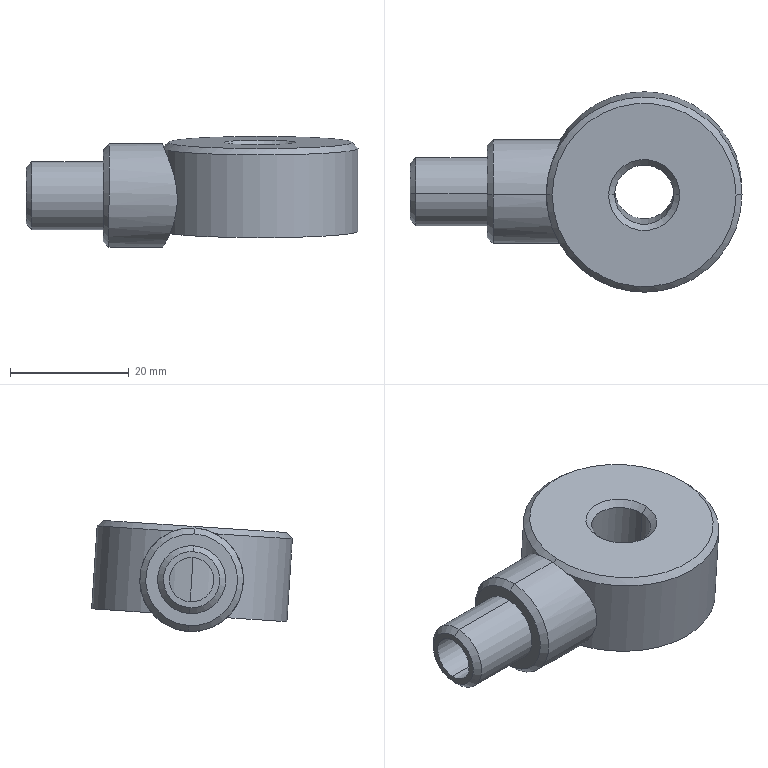Component | SolidWorks | LEDAlarm-1_UpperRotatingHead-1 | 3 solids | 27 faces | box 56 x 33.85 x 18.75 mm | volume 13801 mm3 | cylinder 14 | cone 8 | plane 5 | commonest cylinder face diameters 11.5 x4 33 x4 7.5 x2 17.5 x2 10 x2
build123d program:
from build123d import *

# Parameters (mm, degrees)
SKETCH1_R                = 16.5
SKETCH1_R_2              = 5
BOSS_EXTRUDE1_DEPTH      = 15
CHAMFER1_SIZE            = 1
EXTRUDE_THIN1_REACH      = 50.438
EXTRUDE_THIN1_END_RADIUS = 16.5
SKETCH3_R                = 8.75
SKETCH3_R_2              = 5.75
SKETCH4_R                = 5.75
SKETCH4_R_2              = 3.75
EXTRUDE_THIN2_DEPTH      = 13
CHAMFER2_SIZE            = 1
CHAMFER3_SIZE            = 1


with BuildPart() as part:
    # Sketch1 → Boss-Extrude1 (new body)
    with BuildSketch(Plane.XY):
        Circle(SKETCH1_R)
        Circle(SKETCH1_R_2, mode=Mode.SUBTRACT)
    extrude(amount=BOSS_EXTRUDE1_DEPTH)

    # Chamfer1
    chamfer1_edges = [part.edges().sort_by_distance(p)[0] for p in [
        (-16.5, 0, 15),
        (-5, 0, 15),
    ]]
    chamfer(chamfer1_edges, length=CHAMFER1_SIZE)


with BuildPart() as body_2:
    # Extrude-Thin1: up to this cylinder (the profile starts outside it)
    extrude_thin1_end = Plane(origin=(0, 0, -2.503), z_dir=(0, 0, -1)) * Cylinder(EXTRUDE_THIN1_END_RADIUS, 134.876, mode=Mode.PRIVATE)
    # Sketch3 → Extrude-Thin1 (new, up to the surface)
    with BuildSketch(Plane.ZY.offset(26.5), mode=Mode.PRIVATE) as extrude_thin1_sk1:
        with Locations((6, 0)):
            Circle(SKETCH3_R)
        with Locations((6, 0)):
            Circle(SKETCH3_R_2, mode=Mode.SUBTRACT)
    extrude_thin1_tool1 = extrude(extrude_thin1_sk1.sketch, amount=-EXTRUDE_THIN1_REACH, mode=Mode.PRIVATE) - extrude_thin1_end
    add(extrude_thin1_tool1.solids().sort_by_distance((-26.5, 0, -2.503))[0])

    # Chamfer2
    chamfer2_edges = [body_2.edges().sort_by_distance(p)[0] for p in [
        (-26.5, 0, -2.75),
    ]]
    chamfer(chamfer2_edges, length=CHAMFER2_SIZE)


with BuildPart() as body_3:
    # Sketch4 → Extrude-Thin2 (new body)
    with BuildSketch(Plane.ZY.offset(26.5)):
        with Locations((6, 0)):
            Circle(SKETCH4_R)
        with Locations((6, 0)):
            Circle(SKETCH4_R_2, mode=Mode.SUBTRACT)
    extrude(amount=EXTRUDE_THIN2_DEPTH)

    # Chamfer3
    chamfer3_edges = [body_3.edges().sort_by_distance(p)[0] for p in [
        (-39.5, 0, 0.25),
    ]]
    chamfer(chamfer3_edges, length=CHAMFER3_SIZE)


solid = Compound([part.part, body_2.part, body_3.part])

# Placed as in the assembly
solid = solid.moved(Location((826.947, 455.702, 430.35), (3.768, 0.005615, -0.0003082)))
STEP:
#1=CARTESIAN_POINT('',(31.002,17.913,17.365));
#2=VERTEX_POINT('',#1);
#3=CARTESIAN_POINT('',(31.002,17.938,16.992));
#4=VERTEX_POINT('',#3);
#5=CARTESIAN_POINT('',(31.002,17.925,17.179));
#6=DIRECTION('',(-1.,0.,0.00009864));
#7=DIRECTION('',(0.00009843,-0.06571,0.9978));
#8=AXIS2_PLACEMENT_3D('',#5,#6,#7);
#9=CIRCLE('',#8,0.187);
#10=EDGE_CURVE('',#2,#4,#9,.T.);
#11=ORIENTED_EDGE('',*,*,#10,.F.);
#12=CARTESIAN_POINT('',(31.041,17.911,17.405));
#13=VERTEX_POINT('',#12);
#14=CARTESIAN_POINT('',(31.002,17.913,17.365));
#15=DIRECTION('',(0.7072,-0.04647,0.7055));
#16=VECTOR('',#15,39.37);
#17=LINE('',#14,#16);
#18=EDGE_CURVE('',#2,#13,#17,.T.);
#19=ORIENTED_EDGE('',*,*,#18,.T.);
#20=CARTESIAN_POINT('',(31.041,17.94,16.953));
#21=VERTEX_POINT('',#20);
#22=CARTESIAN_POINT('',(31.041,17.925,17.179));
#23=DIRECTION('',(1.,-0.,-0.00009864));
#24=DIRECTION('',(0.00009843,-0.06571,0.9978));
#25=AXIS2_PLACEMENT_3D('',#22,#23,#24);
#26=CIRCLE('',#25,0.2264);
#27=EDGE_CURVE('',#21,#13,#26,.T.);
#28=ORIENTED_EDGE('',*,*,#27,.F.);
#29=CARTESIAN_POINT('',(31.002,17.938,16.992));
#30=DIRECTION('',(0.707,0.04647,-0.7056));
#31=VECTOR('',#30,39.37);
#32=LINE('',#29,#31);
#33=EDGE_CURVE('',#4,#21,#32,.T.);
#34=ORIENTED_EDGE('',*,*,#33,.F.);
#35=EDGE_LOOP('',(#11,#19,#28,#34));
#36=FACE_OUTER_BOUND('',#35,.T.);
#37=CARTESIAN_POINT('',(31.002,17.925,17.179));
#38=DIRECTION('',(1.,-0.,-0.00009864));
#39=DIRECTION('',(-0.00009843,0.06571,-0.9978));
#40=AXIS2_PLACEMENT_3D('',#37,#38,#39);
#41=CONICAL_SURFACE('',#40,0.187,0.7854);
#42=ADVANCED_FACE('',(#36),#41,.T.);
#43=CARTESIAN_POINT('',(31.002,17.935,17.031));
#44=VERTEX_POINT('',#43);
#45=CARTESIAN_POINT('',(31.002,17.916,17.326));
#46=VERTEX_POINT('',#45);
#47=CARTESIAN_POINT('',(31.002,17.925,17.179));
#48=DIRECTION('',(-1.,0.,0.00009864));
#49=DIRECTION('',(0.00009843,-0.06571,0.9978));
#50=AXIS2_PLACEMENT_3D('',#47,#48,#49);
#51=CIRCLE('',#50,0.1476);
#52=EDGE_CURVE('',#44,#46,#51,.T.);
#53=ORIENTED_EDGE('',*,*,#52,.T.);
#54=CARTESIAN_POINT('',(31.514,17.916,17.326));
#55=VERTEX_POINT('',#54);
#56=CARTESIAN_POINT('',(31.002,17.916,17.326));
#57=DIRECTION('',(1.,-0.,-0.00009864));
#58=VECTOR('',#57,39.37);
#59=LINE('',#56,#58);
#60=EDGE_CURVE('',#46,#55,#59,.T.);
#61=ORIENTED_EDGE('',*,*,#60,.T.);
#62=CARTESIAN_POINT('',(31.514,17.935,17.031));
#63=VERTEX_POINT('',#62);
#64=CARTESIAN_POINT('',(31.514,17.925,17.179));
#65=DIRECTION('',(-1.,0.,0.00009864));
#66=DIRECTION('',(0.00009843,-0.06571,0.9978));
#67=AXIS2_PLACEMENT_3D('',#64,#65,#66);
#68=CIRCLE('',#67,0.1476);
#69=EDGE_CURVE('',#63,#55,#68,.T.);
#70=ORIENTED_EDGE('',*,*,#69,.F.);
#71=CARTESIAN_POINT('',(31.002,17.935,17.031));
#72=DIRECTION('',(1.,-0.,-0.00009864));
#73=VECTOR('',#72,39.37);
#74=LINE('',#71,#73);
#75=EDGE_CURVE('',#44,#63,#74,.T.);
#76=ORIENTED_EDGE('',*,*,#75,.F.);
#77=EDGE_LOOP('',(#53,#61,#70,#76));
#78=FACE_OUTER_BOUND('',#77,.T.);
#79=CARTESIAN_POINT('',(31.002,17.925,17.179));
#80=DIRECTION('',(1.,-0.,-0.00009864));
#81=DIRECTION('',(-0.00009843,0.06571,-0.9978));
#82=AXIS2_PLACEMENT_3D('',#79,#80,#81);
#83=CYLINDRICAL_SURFACE('',#82,0.1476);
#84=ADVANCED_FACE('',(#78),#83,.F.);
#85=ORIENTED_EDGE('',*,*,#27,.T.);
#86=CARTESIAN_POINT('',(31.514,17.911,17.405));
#87=VERTEX_POINT('',#86);
#88=CARTESIAN_POINT('',(31.002,17.911,17.405));
#89=DIRECTION('',(1.,-0.,-0.00009864));
#90=VECTOR('',#89,39.37);
#91=LINE('',#88,#90);
#92=EDGE_CURVE('',#13,#87,#91,.T.);
#93=ORIENTED_EDGE('',*,*,#92,.T.);
#94=CARTESIAN_POINT('',(31.514,17.94,16.953));
#95=VERTEX_POINT('',#94);
#96=CARTESIAN_POINT('',(31.514,17.925,17.179));
#97=DIRECTION('',(-1.,0.,0.00009864));
#98=DIRECTION('',(0.00009843,-0.06571,0.9978));
#99=AXIS2_PLACEMENT_3D('',#96,#97,#98);
#100=CIRCLE('',#99,0.2264);
#101=EDGE_CURVE('',#87,#95,#100,.T.);
#102=ORIENTED_EDGE('',*,*,#101,.T.);
#103=CARTESIAN_POINT('',(31.002,17.94,16.953));
#104=DIRECTION('',(1.,-0.,-0.00009864));
#105=VECTOR('',#104,39.37);
#106=LINE('',#103,#105);
#107=EDGE_CURVE('',#21,#95,#106,.T.);
#108=ORIENTED_EDGE('',*,*,#107,.F.);
#109=EDGE_LOOP('',(#85,#93,#102,#108));
#110=FACE_OUTER_BOUND('',#109,.T.);
#111=CARTESIAN_POINT('',(31.002,17.925,17.179));
#112=DIRECTION('',(1.,-0.,-0.00009864));
#113=DIRECTION('',(-0.00009843,0.06571,-0.9978));
#114=AXIS2_PLACEMENT_3D('',#111,#112,#113);
#115=CYLINDRICAL_SURFACE('',#114,0.2264);
#116=ADVANCED_FACE('',(#110),#115,.T.);
#117=CARTESIAN_POINT('',(31.002,17.925,17.179));
#118=DIRECTION('',(-1.,0.,0.00009864));
#119=DIRECTION('',(0.00009843,-0.06571,0.9978));
#120=AXIS2_PLACEMENT_3D('',#117,#118,#119);
#121=CIRCLE('',#120,0.187);
#122=EDGE_CURVE('',#4,#2,#121,.T.);
#123=ORIENTED_EDGE('',*,*,#122,.T.);
#124=ORIENTED_EDGE('',*,*,#10,.T.);
#125=EDGE_LOOP('',(#123,#124));
#126=FACE_OUTER_BOUND('',#125,.T.);
#127=ORIENTED_EDGE('',*,*,#52,.F.);
#128=CARTESIAN_POINT('',(31.002,17.925,17.179));
#129=DIRECTION('',(-1.,0.,0.00009864));
#130=DIRECTION('',(0.00009843,-0.06571,0.9978));
#131=AXIS2_PLACEMENT_3D('',#128,#129,#130);
#132=CIRCLE('',#131,0.1476);
#133=EDGE_CURVE('',#46,#44,#132,.T.);
#134=ORIENTED_EDGE('',*,*,#133,.F.);
#135=EDGE_LOOP('',(#127,#134));
#136=FACE_BOUND('',#135,.T.);
#137=CARTESIAN_POINT('',(31.002,17.925,17.179));
#138=DIRECTION('',(-1.,0.,0.00009864));
#139=DIRECTION('',(0.00009843,-0.06571,0.9978));
#140=AXIS2_PLACEMENT_3D('',#137,#138,#139);
#141=PLANE('',#140);
#142=ADVANCED_FACE('',(#126,#136),#141,.T.);
#143=CARTESIAN_POINT('',(31.514,17.925,17.179));
#144=DIRECTION('',(-1.,0.,0.00009864));
#145=DIRECTION('',(0.00009843,-0.06571,0.9978));
#146=AXIS2_PLACEMENT_3D('',#143,#144,#145);
#147=CIRCLE('',#146,0.2264);
#148=EDGE_CURVE('',#95,#87,#147,.T.);
#149=ORIENTED_EDGE('',*,*,#148,.F.);
#150=ORIENTED_EDGE('',*,*,#101,.F.);
#151=EDGE_LOOP('',(#149,#150));
#152=FACE_OUTER_BOUND('',#151,.T.);
#153=ORIENTED_EDGE('',*,*,#69,.T.);
#154=CARTESIAN_POINT('',(31.514,17.925,17.179));
#155=DIRECTION('',(-1.,0.,0.00009864));
#156=DIRECTION('',(0.00009843,-0.06571,0.9978));
#157=AXIS2_PLACEMENT_3D('',#154,#155,#156);
#158=CIRCLE('',#157,0.1476);
#159=EDGE_CURVE('',#55,#63,#158,.T.);
#160=ORIENTED_EDGE('',*,*,#159,.T.);
#161=EDGE_LOOP('',(#153,#160));
#162=FACE_BOUND('',#161,.T.);
#163=CARTESIAN_POINT('',(31.514,17.925,17.179));
#164=DIRECTION('',(-1.,0.,0.00009864));
#165=DIRECTION('',(0.00009843,-0.06571,0.9978));
#166=AXIS2_PLACEMENT_3D('',#163,#164,#165);
#167=PLANE('',#166);
#168=ADVANCED_FACE('',(#152,#162),#167,.F.);
#169=ORIENTED_EDGE('',*,*,#92,.F.);
#170=CARTESIAN_POINT('',(31.041,17.925,17.179));
#171=DIRECTION('',(1.,-0.,-0.00009864));
#172=DIRECTION('',(0.00009843,-0.06571,0.9978));
#173=AXIS2_PLACEMENT_3D('',#170,#171,#172);
#174=CIRCLE('',#173,0.2264);
#175=EDGE_CURVE('',#13,#21,#174,.T.);
#176=ORIENTED_EDGE('',*,*,#175,.T.);
#177=ORIENTED_EDGE('',*,*,#107,.T.);
#178=ORIENTED_EDGE('',*,*,#148,.T.);
#179=EDGE_LOOP('',(#169,#176,#177,#178));
#180=FACE_OUTER_BOUND('',#179,.T.);
#181=CARTESIAN_POINT('',(31.002,17.925,17.179));
#182=DIRECTION('',(1.,-0.,-0.00009864));
#183=DIRECTION('',(-0.00009843,0.06571,-0.9978));
#184=AXIS2_PLACEMENT_3D('',#181,#182,#183);
#185=CYLINDRICAL_SURFACE('',#184,0.2264);
#186=ADVANCED_FACE('',(#180),#185,.T.);
#187=ORIENTED_EDGE('',*,*,#60,.F.);
#188=ORIENTED_EDGE('',*,*,#133,.T.);
#189=ORIENTED_EDGE('',*,*,#75,.T.);
#190=ORIENTED_EDGE('',*,*,#159,.F.);
#191=EDGE_LOOP('',(#187,#188,#189,#190));
#192=FACE_OUTER_BOUND('',#191,.T.);
#193=CARTESIAN_POINT('',(31.002,17.925,17.179));
#194=DIRECTION('',(1.,-0.,-0.00009864));
#195=DIRECTION('',(-0.00009843,0.06571,-0.9978));
#196=AXIS2_PLACEMENT_3D('',#193,#194,#195);
#197=CYLINDRICAL_SURFACE('',#196,0.1476);
#198=ADVANCED_FACE('',(#192),#197,.F.);
#199=ORIENTED_EDGE('',*,*,#18,.F.);
#200=ORIENTED_EDGE('',*,*,#122,.F.);
#201=ORIENTED_EDGE('',*,*,#33,.T.);
#202=ORIENTED_EDGE('',*,*,#175,.F.);
#203=EDGE_LOOP('',(#199,#200,#201,#202));
#204=FACE_OUTER_BOUND('',#203,.T.);
#205=CARTESIAN_POINT('',(31.002,17.925,17.179));
#206=DIRECTION('',(1.,-0.,-0.00009864));
#207=DIRECTION('',(-0.00009843,0.06571,-0.9978));
#208=AXIS2_PLACEMENT_3D('',#205,#206,#207);
#209=CONICAL_SURFACE('',#208,0.187,0.7854);
#210=ADVANCED_FACE('',(#204),#209,.T.);
#211=CLOSED_SHELL('',(#42,#84,#116,#142,#168,#186,#198,#210));
#212=MANIFOLD_SOLID_BREP('',#211);
#213=CARTESIAN_POINT('',(31.514,17.905,17.483));
#214=VERTEX_POINT('',#213);
#215=CARTESIAN_POINT('',(31.514,17.946,16.874));
#216=VERTEX_POINT('',#215);
#217=CARTESIAN_POINT('',(31.514,17.925,17.179));
#218=DIRECTION('',(-1.,0.,0.00009864));
#219=DIRECTION('',(0.00009843,-0.06571,0.9978));
#220=AXIS2_PLACEMENT_3D('',#217,#218,#219);
#221=CIRCLE('',#220,0.3051);
#222=EDGE_CURVE('',#214,#216,#221,.T.);
#223=ORIENTED_EDGE('',*,*,#222,.F.);
#224=CARTESIAN_POINT('',(31.553,17.903,17.522));
#225=VERTEX_POINT('',#224);
#226=CARTESIAN_POINT('',(31.514,17.905,17.483));
#227=DIRECTION('',(0.7072,-0.04647,0.7055));
#228=VECTOR('',#227,39.37);
#229=LINE('',#226,#228);
#230=EDGE_CURVE('',#214,#225,#229,.T.);
#231=ORIENTED_EDGE('',*,*,#230,.T.);
#232=CARTESIAN_POINT('',(31.553,17.948,16.835));
#233=VERTEX_POINT('',#232);
#234=CARTESIAN_POINT('',(31.553,17.925,17.179));
#235=DIRECTION('',(1.,-0.,-0.00009864));
#236=DIRECTION('',(0.00009843,-0.06571,0.9978));
#237=AXIS2_PLACEMENT_3D('',#234,#235,#236);
#238=CIRCLE('',#237,0.3445);
#239=EDGE_CURVE('',#233,#225,#238,.T.);
#240=ORIENTED_EDGE('',*,*,#239,.F.);
#241=CARTESIAN_POINT('',(31.514,17.946,16.874));
#242=DIRECTION('',(0.707,0.04647,-0.7056));
#243=VECTOR('',#242,39.37);
#244=LINE('',#241,#243);
#245=EDGE_CURVE('',#216,#233,#244,.T.);
#246=ORIENTED_EDGE('',*,*,#245,.F.);
#247=EDGE_LOOP('',(#223,#231,#240,#246));
#248=FACE_OUTER_BOUND('',#247,.T.);
#249=CARTESIAN_POINT('',(31.514,17.925,17.179));
#250=DIRECTION('',(1.,-0.,-0.00009864));
#251=DIRECTION('',(-0.00009843,0.06571,-0.9978));
#252=AXIS2_PLACEMENT_3D('',#249,#250,#251);
#253=CONICAL_SURFACE('',#252,0.3051,0.7854);
#254=ADVANCED_FACE('',(#248),#253,.T.);
#255=CARTESIAN_POINT('',(31.907,17.94,16.953));
#256=VERTEX_POINT('',#255);
#257=CARTESIAN_POINT('',(31.907,17.911,17.405));
#258=VERTEX_POINT('',#257);
#259=CARTESIAN_POINT('',(31.907,17.94,16.953));
#260=CARTESIAN_POINT('',(31.907,17.933,16.952));
#261=CARTESIAN_POINT('',(31.908,17.926,16.952));
#262=CARTESIAN_POINT('',(31.908,17.911,16.953));
#263=CARTESIAN_POINT('',(31.908,17.903,16.953));
#264=CARTESIAN_POINT('',(31.91,17.881,16.956));
#265=CARTESIAN_POINT('',(31.911,17.866,16.96));
#266=CARTESIAN_POINT('',(31.915,17.838,16.969));
#267=CARTESIAN_POINT('',(31.917,17.825,16.975));
#268=CARTESIAN_POINT('',(31.922,17.799,16.99));
#269=CARTESIAN_POINT('',(31.925,17.787,16.999));
#270=CARTESIAN_POINT('',(31.93,17.765,17.018));
#271=CARTESIAN_POINT('',(31.933,17.755,17.029));
#272=CARTESIAN_POINT('',(31.936,17.742,17.046));
#273=CARTESIAN_POINT('',(31.938,17.737,17.052));
#274=CARTESIAN_POINT('',(31.94,17.73,17.065));
#275=CARTESIAN_POINT('',(31.941,17.726,17.072));
#276=CARTESIAN_POINT('',(31.944,17.716,17.092));
#277=CARTESIAN_POINT('',(31.945,17.711,17.105));
#278=CARTESIAN_POINT('',(31.948,17.703,17.134));
#279=CARTESIAN_POINT('',(31.948,17.701,17.149));
#280=CARTESIAN_POINT('',(31.948,17.699,17.179));
#281=CARTESIAN_POINT('',(31.948,17.699,17.194));
#282=CARTESIAN_POINT('',(31.946,17.702,17.216));
#283=CARTESIAN_POINT('',(31.945,17.703,17.223));
#284=CARTESIAN_POINT('',(31.944,17.707,17.238));
#285=CARTESIAN_POINT('',(31.943,17.709,17.245));
#286=CARTESIAN_POINT('',(31.941,17.714,17.259));
#287=CARTESIAN_POINT('',(31.94,17.716,17.266));
#288=CARTESIAN_POINT('',(31.938,17.722,17.279));
#289=CARTESIAN_POINT('',(31.936,17.726,17.286));
#290=CARTESIAN_POINT('',(31.933,17.737,17.305));
#291=CARTESIAN_POINT('',(31.93,17.746,17.317));
#292=CARTESIAN_POINT('',(31.925,17.765,17.339));
#293=CARTESIAN_POINT('',(31.922,17.776,17.349));
#294=CARTESIAN_POINT('',(31.917,17.799,17.367));
#295=CARTESIAN_POINT('',(31.915,17.812,17.375));
#296=CARTESIAN_POINT('',(31.912,17.832,17.385));
#297=CARTESIAN_POINT('',(31.912,17.838,17.388));
#298=CARTESIAN_POINT('',(31.91,17.852,17.393));
#299=CARTESIAN_POINT('',(31.909,17.859,17.395));
#300=CARTESIAN_POINT('',(31.908,17.881,17.401));
#301=CARTESIAN_POINT('',(31.907,17.896,17.404));
#302=CARTESIAN_POINT('',(31.907,17.911,17.405));
#303=B_SPLINE_CURVE_WITH_KNOTS('',3,(#259,#260,#261,#262,#263,#264,#265,#266,#267,#268,#269,#270,#271,#272,#273,#274,#275,#276,#277,#278,#279,#280,#281,#282,#283,#284,#285,#286,#287,#288,#289,#290,#291,#292,#293,#294,#295,#296,#297,#298,#299,#300,#301,#302),.UNSPECIFIED.,.F.,.F.,(4,2,2,2,2,2,2,2,2,2,2,2,2,2,2,2,2,2,2,2,2,4),(0.01812,0.01869,0.01925,0.02038,0.02152,0.02265,0.02378,0.02435,0.02491,0.02605,0.02718,0.02831,0.02888,0.02944,0.03001,0.03058,0.03171,0.03284,0.03397,0.03454,0.0351,0.03624),.UNSPECIFIED.);
#304=EDGE_CURVE('',#256,#258,#303,.T.);
#305=ORIENTED_EDGE('',*,*,#304,.F.);
#306=CARTESIAN_POINT('',(31.514,17.94,16.953));
#307=VERTEX_POINT('',#306);
#308=CARTESIAN_POINT('',(33.207,17.94,16.953));
#309=DIRECTION('',(-1.,0.,0.00009864));
#310=VECTOR('',#309,39.37);
#311=LINE('',#308,#310);
#312=EDGE_CURVE('',#256,#307,#311,.T.);
#313=ORIENTED_EDGE('',*,*,#312,.T.);
#314=CARTESIAN_POINT('',(31.514,17.911,17.405));
#315=VERTEX_POINT('',#314);
#316=CARTESIAN_POINT('',(31.514,17.925,17.179));
#317=DIRECTION('',(-1.,0.,0.00009864));
#318=DIRECTION('',(0.00009843,-0.06571,0.9978));
#319=AXIS2_PLACEMENT_3D('',#316,#317,#318);
#320=CIRCLE('',#319,0.2264);
#321=EDGE_CURVE('',#307,#315,#320,.T.);
#322=ORIENTED_EDGE('',*,*,#321,.T.);
#323=CARTESIAN_POINT('',(33.207,17.911,17.404));
#324=DIRECTION('',(-1.,0.,0.00009864));
#325=VECTOR('',#324,39.37);
#326=LINE('',#323,#325);
#327=EDGE_CURVE('',#258,#315,#326,.T.);
#328=ORIENTED_EDGE('',*,*,#327,.F.);
#329=EDGE_LOOP('',(#305,#313,#322,#328));
#330=FACE_OUTER_BOUND('',#329,.T.);
#331=CARTESIAN_POINT('',(33.207,17.925,17.179));
#332=DIRECTION('',(-1.,0.,0.00009864));
#333=DIRECTION('',(0.00009843,-0.06571,0.9978));
#334=AXIS2_PLACEMENT_3D('',#331,#332,#333);
#335=CYLINDRICAL_SURFACE('',#334,0.2264);
#336=ADVANCED_FACE('',(#330),#335,.F.);
#337=CARTESIAN_POINT('',(31.907,17.903,17.522));
#338=VERTEX_POINT('',#337);
#339=CARTESIAN_POINT('',(31.907,17.948,16.835));
#340=VERTEX_POINT('',#339);
#341=CARTESIAN_POINT('',(31.907,17.903,17.522));
#342=CARTESIAN_POINT('',(31.907,17.926,17.524));
#343=CARTESIAN_POINT('',(31.909,17.949,17.523));
#344=CARTESIAN_POINT('',(31.913,17.994,17.517));
#345=CARTESIAN_POINT('',(31.917,18.017,17.512));
#346=CARTESIAN_POINT('',(31.926,18.059,17.497));
#347=CARTESIAN_POINT('',(31.931,18.08,17.488));
#348=CARTESIAN_POINT('',(31.94,18.109,17.471));
#349=CARTESIAN_POINT('',(31.943,18.118,17.465));
#350=CARTESIAN_POINT('',(31.949,18.136,17.452));
#351=CARTESIAN_POINT('',(31.952,18.145,17.445));
#352=CARTESIAN_POINT('',(31.958,18.161,17.43));
#353=CARTESIAN_POINT('',(31.961,18.169,17.423));
#354=CARTESIAN_POINT('',(31.968,18.184,17.406));
#355=CARTESIAN_POINT('',(31.971,18.192,17.398));
#356=CARTESIAN_POINT('',(31.98,18.212,17.371));
#357=CARTESIAN_POINT('',(31.986,18.224,17.353));
#358=CARTESIAN_POINT('',(31.993,18.239,17.323));
#359=CARTESIAN_POINT('',(31.995,18.243,17.312));
#360=CARTESIAN_POINT('',(31.999,18.251,17.291));
#361=CARTESIAN_POINT('',(32.001,18.255,17.28));
#362=CARTESIAN_POINT('',(32.005,18.264,17.247));
#363=CARTESIAN_POINT('',(32.006,18.268,17.225));
#364=CARTESIAN_POINT('',(32.006,18.27,17.19));
#365=CARTESIAN_POINT('',(32.006,18.27,17.179));
#366=CARTESIAN_POINT('',(32.004,18.269,17.156));
#367=CARTESIAN_POINT('',(32.003,18.268,17.144));
#368=CARTESIAN_POINT('',(32.001,18.265,17.122));
#369=CARTESIAN_POINT('',(31.999,18.263,17.11));
#370=CARTESIAN_POINT('',(31.995,18.258,17.088));
#371=CARTESIAN_POINT('',(31.993,18.255,17.077));
#372=CARTESIAN_POINT('',(31.985,18.244,17.045));
#373=CARTESIAN_POINT('',(31.98,18.235,17.025));
#374=CARTESIAN_POINT('',(31.971,18.218,16.996));
#375=CARTESIAN_POINT('',(31.967,18.212,16.987));
#376=CARTESIAN_POINT('',(31.961,18.199,16.969));
#377=CARTESIAN_POINT('',(31.958,18.192,16.96));
#378=CARTESIAN_POINT('',(31.949,18.17,16.935));
#379=CARTESIAN_POINT('',(31.942,18.154,16.92));
#380=CARTESIAN_POINT('',(31.931,18.118,16.892));
#381=CARTESIAN_POINT('',(31.926,18.1,16.881));
#382=CARTESIAN_POINT('',(31.919,18.069,16.866));
#383=CARTESIAN_POINT('',(31.917,18.059,16.861));
#384=CARTESIAN_POINT('',(31.914,18.038,16.853));
#385=CARTESIAN_POINT('',(31.912,18.027,16.849));
#386=CARTESIAN_POINT('',(31.909,17.994,16.84));
#387=CARTESIAN_POINT('',(31.907,17.971,16.836));
#388=CARTESIAN_POINT('',(31.907,17.948,16.835));
#389=B_SPLINE_CURVE_WITH_KNOTS('',3,(#341,#342,#343,#344,#345,#346,#347,#348,#349,#350,#351,#352,#353,#354,#355,#356,#357,#358,#359,#360,#361,#362,#363,#364,#365,#366,#367,#368,#369,#370,#371,#372,#373,#374,#375,#376,#377,#378,#379,#380,#381,#382,#383,#384,#385,#386,#387,#388),.UNSPECIFIED.,.F.,.F.,(4,2,2,2,2,2,2,2,2,2,2,2,2,2,2,2,2,2,2,2,2,2,2,4),(0.,0.001744,0.003488,0.005232,0.006103,0.006975,0.007847,0.008719,0.01046,0.01133,0.01221,0.01395,0.01482,0.01569,0.01657,0.01744,0.01918,0.02005,0.02093,0.02267,0.02441,0.02529,0.02616,0.0279),.UNSPECIFIED.);
#390=EDGE_CURVE('',#338,#340,#389,.T.);
#391=ORIENTED_EDGE('',*,*,#390,.T.);
#392=CARTESIAN_POINT('',(33.207,17.948,16.835));
#393=DIRECTION('',(-1.,0.,0.00009864));
#394=VECTOR('',#393,39.37);
#395=LINE('',#392,#394);
#396=EDGE_CURVE('',#340,#233,#395,.T.);
#397=ORIENTED_EDGE('',*,*,#396,.T.);
#398=ORIENTED_EDGE('',*,*,#239,.T.);
#399=CARTESIAN_POINT('',(33.207,17.903,17.522));
#400=DIRECTION('',(-1.,0.,0.00009864));
#401=VECTOR('',#400,39.37);
#402=LINE('',#399,#401);
#403=EDGE_CURVE('',#338,#225,#402,.T.);
#404=ORIENTED_EDGE('',*,*,#403,.F.);
#405=EDGE_LOOP('',(#391,#397,#398,#404));
#406=FACE_OUTER_BOUND('',#405,.T.);
#407=CARTESIAN_POINT('',(33.207,17.925,17.179));
#408=DIRECTION('',(-1.,0.,0.00009864));
#409=DIRECTION('',(0.00009843,-0.06571,0.9978));
#410=AXIS2_PLACEMENT_3D('',#407,#408,#409);
#411=CYLINDRICAL_SURFACE('',#410,0.3445);
#412=ADVANCED_FACE('',(#406),#411,.T.);
#413=ORIENTED_EDGE('',*,*,#390,.F.);
#414=CARTESIAN_POINT('',(31.907,17.902,17.532));
#415=DIRECTION('',(-0.00009843,0.06571,-0.9978));
#416=VECTOR('',#415,39.37);
#417=LINE('',#414,#416);
#418=EDGE_CURVE('',#338,#258,#417,.T.);
#419=ORIENTED_EDGE('',*,*,#418,.T.);
#420=CARTESIAN_POINT('',(31.907,17.911,17.405));
#421=CARTESIAN_POINT('',(31.907,17.926,17.406));
#422=CARTESIAN_POINT('',(31.908,17.941,17.405));
#423=CARTESIAN_POINT('',(31.909,17.963,17.402));
#424=CARTESIAN_POINT('',(31.91,17.97,17.401));
#425=CARTESIAN_POINT('',(31.912,17.984,17.397));
#426=CARTESIAN_POINT('',(31.912,17.992,17.395));
#427=CARTESIAN_POINT('',(31.915,18.013,17.388));
#428=CARTESIAN_POINT('',(31.917,18.026,17.382));
#429=CARTESIAN_POINT('',(31.921,18.045,17.371));
#430=CARTESIAN_POINT('',(31.922,18.052,17.367));
#431=CARTESIAN_POINT('',(31.925,18.064,17.358));
#432=CARTESIAN_POINT('',(31.926,18.069,17.354));
#433=CARTESIAN_POINT('',(31.93,18.086,17.339));
#434=CARTESIAN_POINT('',(31.933,18.096,17.329));
#435=CARTESIAN_POINT('',(31.938,18.114,17.305));
#436=CARTESIAN_POINT('',(31.94,18.122,17.292));
#437=CARTESIAN_POINT('',(31.943,18.132,17.273));
#438=CARTESIAN_POINT('',(31.944,18.135,17.266));
#439=CARTESIAN_POINT('',(31.945,18.14,17.252));
#440=CARTESIAN_POINT('',(31.946,18.142,17.245));
#441=CARTESIAN_POINT('',(31.948,18.148,17.223));
#442=CARTESIAN_POINT('',(31.948,18.15,17.209));
#443=CARTESIAN_POINT('',(31.948,18.152,17.179));
#444=CARTESIAN_POINT('',(31.948,18.152,17.164));
#445=CARTESIAN_POINT('',(31.945,18.148,17.134));
#446=CARTESIAN_POINT('',(31.944,18.145,17.12));
#447=CARTESIAN_POINT('',(31.94,18.135,17.091));
#448=CARTESIAN_POINT('',(31.938,18.129,17.078));
#449=CARTESIAN_POINT('',(31.934,18.118,17.059));
#450=CARTESIAN_POINT('',(31.933,18.114,17.053));
#451=CARTESIAN_POINT('',(31.93,18.105,17.041));
#452=CARTESIAN_POINT('',(31.929,18.101,17.035));
#453=CARTESIAN_POINT('',(31.925,18.086,17.018));
#454=CARTESIAN_POINT('',(31.922,18.075,17.008));
#455=CARTESIAN_POINT('',(31.917,18.052,16.99));
#456=CARTESIAN_POINT('',(31.915,18.039,16.982));
#457=CARTESIAN_POINT('',(31.911,18.013,16.969));
#458=CARTESIAN_POINT('',(31.91,17.999,16.964));
#459=CARTESIAN_POINT('',(31.908,17.977,16.958));
#460=CARTESIAN_POINT('',(31.908,17.97,16.957));
#461=CARTESIAN_POINT('',(31.908,17.955,16.954));
#462=CARTESIAN_POINT('',(31.907,17.948,16.953));
#463=CARTESIAN_POINT('',(31.907,17.94,16.953));
#464=B_SPLINE_CURVE_WITH_KNOTS('',3,(#420,#421,#422,#423,#424,#425,#426,#427,#428,#429,#430,#431,#432,#433,#434,#435,#436,#437,#438,#439,#440,#441,#442,#443,#444,#445,#446,#447,#448,#449,#450,#451,#452,#453,#454,#455,#456,#457,#458,#459,#460,#461,#462,#463),.UNSPECIFIED.,.F.,.F.,(4,2,2,2,2,2,2,2,2,2,2,2,2,2,2,2,2,2,2,2,2,4),(0.,0.001133,0.001699,0.002265,0.003398,0.003964,0.00453,0.005663,0.006795,0.007361,0.007928,0.00906,0.01019,0.01133,0.01246,0.01302,0.01359,0.01472,0.01586,0.01699,0.01755,0.01812),.UNSPECIFIED.);
#465=EDGE_CURVE('',#258,#256,#464,.T.);
#466=ORIENTED_EDGE('',*,*,#465,.T.);
#467=CARTESIAN_POINT('',(31.907,17.902,17.532));
#468=DIRECTION('',(-0.00009843,0.06571,-0.9978));
#469=VECTOR('',#468,39.37);
#470=LINE('',#467,#469);
#471=EDGE_CURVE('',#256,#340,#470,.T.);
#472=ORIENTED_EDGE('',*,*,#471,.T.);
#473=EDGE_LOOP('',(#413,#419,#466,#472));
#474=FACE_OUTER_BOUND('',#473,.T.);
#475=CARTESIAN_POINT('',(32.557,17.902,17.532));
#476=DIRECTION('',(-0.00009843,0.06571,-0.9978));
#477=DIRECTION('',(-1.,0.,0.00009864));
#478=AXIS2_PLACEMENT_3D('',#475,#476,#477);
#479=CYLINDRICAL_SURFACE('',#478,0.6496);
#480=ADVANCED_FACE('',(#474),#479,.F.);
#481=ORIENTED_EDGE('',*,*,#418,.F.);
#482=CARTESIAN_POINT('',(31.907,17.948,16.835));
#483=CARTESIAN_POINT('',(31.907,17.937,16.834));
#484=CARTESIAN_POINT('',(31.908,17.925,16.834));
#485=CARTESIAN_POINT('',(31.909,17.902,16.835));
#486=CARTESIAN_POINT('',(31.91,17.891,16.836));
#487=CARTESIAN_POINT('',(31.913,17.857,16.84));
#488=CARTESIAN_POINT('',(31.917,17.835,16.846));
#489=CARTESIAN_POINT('',(31.926,17.792,16.86));
#490=CARTESIAN_POINT('',(31.931,17.771,16.87));
#491=CARTESIAN_POINT('',(31.942,17.733,16.892));
#492=CARTESIAN_POINT('',(31.949,17.715,16.905));
#493=CARTESIAN_POINT('',(31.961,17.681,16.935));
#494=CARTESIAN_POINT('',(31.968,17.666,16.951));
#495=CARTESIAN_POINT('',(31.977,17.646,16.977));
#496=CARTESIAN_POINT('',(31.98,17.64,16.986));
#497=CARTESIAN_POINT('',(31.985,17.628,17.005));
#498=CARTESIAN_POINT('',(31.988,17.622,17.015));
#499=CARTESIAN_POINT('',(31.995,17.607,17.045));
#500=CARTESIAN_POINT('',(31.999,17.599,17.066));
#501=CARTESIAN_POINT('',(32.005,17.587,17.11));
#502=CARTESIAN_POINT('',(32.006,17.583,17.133));
#503=CARTESIAN_POINT('',(32.006,17.581,17.167));
#504=CARTESIAN_POINT('',(32.006,17.581,17.178));
#505=CARTESIAN_POINT('',(32.005,17.582,17.201));
#506=CARTESIAN_POINT('',(32.003,17.583,17.213));
#507=CARTESIAN_POINT('',(31.999,17.587,17.247));
#508=CARTESIAN_POINT('',(31.995,17.592,17.269));
#509=CARTESIAN_POINT('',(31.988,17.603,17.301));
#510=CARTESIAN_POINT('',(31.985,17.607,17.312));
#511=CARTESIAN_POINT('',(31.98,17.617,17.332));
#512=CARTESIAN_POINT('',(31.977,17.622,17.342));
#513=CARTESIAN_POINT('',(31.971,17.633,17.361));
#514=CARTESIAN_POINT('',(31.968,17.639,17.37));
#515=CARTESIAN_POINT('',(31.961,17.652,17.388));
#516=CARTESIAN_POINT('',(31.958,17.659,17.397));
#517=CARTESIAN_POINT('',(31.949,17.681,17.422));
#518=CARTESIAN_POINT('',(31.942,17.697,17.437));
#519=CARTESIAN_POINT('',(31.934,17.723,17.458));
#520=CARTESIAN_POINT('',(31.931,17.732,17.464));
#521=CARTESIAN_POINT('',(31.926,17.751,17.476));
#522=CARTESIAN_POINT('',(31.924,17.761,17.482));
#523=CARTESIAN_POINT('',(31.917,17.791,17.497));
#524=CARTESIAN_POINT('',(31.914,17.812,17.505));
#525=CARTESIAN_POINT('',(31.91,17.846,17.514));
#526=CARTESIAN_POINT('',(31.909,17.857,17.516));
#527=CARTESIAN_POINT('',(31.908,17.88,17.52));
#528=CARTESIAN_POINT('',(31.907,17.891,17.522));
#529=CARTESIAN_POINT('',(31.907,17.903,17.522));
#530=B_SPLINE_CURVE_WITH_KNOTS('',3,(#482,#483,#484,#485,#486,#487,#488,#489,#490,#491,#492,#493,#494,#495,#496,#497,#498,#499,#500,#501,#502,#503,#504,#505,#506,#507,#508,#509,#510,#511,#512,#513,#514,#515,#516,#517,#518,#519,#520,#521,#522,#523,#524,#525,#526,#527,#528,#529),.UNSPECIFIED.,.F.,.F.,(4,2,2,2,2,2,2,2,2,2,2,2,2,2,2,2,2,2,2,2,2,2,2,4),(0.0279,0.02877,0.02964,0.03138,0.03312,0.03486,0.0366,0.03747,0.03834,0.04008,0.04182,0.04269,0.04356,0.0453,0.04617,0.04704,0.04791,0.04878,0.05052,0.05139,0.05226,0.054,0.05487,0.05574),.UNSPECIFIED.);
#531=EDGE_CURVE('',#340,#338,#530,.T.);
#532=ORIENTED_EDGE('',*,*,#531,.F.);
#533=ORIENTED_EDGE('',*,*,#471,.F.);
#534=ORIENTED_EDGE('',*,*,#304,.T.);
#535=EDGE_LOOP('',(#481,#532,#533,#534));
#536=FACE_OUTER_BOUND('',#535,.T.);
#537=CARTESIAN_POINT('',(32.557,17.902,17.532));
#538=DIRECTION('',(-0.00009843,0.06571,-0.9978));
#539=DIRECTION('',(-1.,0.,0.00009864));
#540=AXIS2_PLACEMENT_3D('',#537,#538,#539);
#541=CYLINDRICAL_SURFACE('',#540,0.6496);
#542=ADVANCED_FACE('',(#536),#541,.F.);
#543=ORIENTED_EDGE('',*,*,#396,.F.);
#544=ORIENTED_EDGE('',*,*,#531,.T.);
#545=ORIENTED_EDGE('',*,*,#403,.T.);
#546=CARTESIAN_POINT('',(31.553,17.925,17.179));
#547=DIRECTION('',(1.,-0.,-0.00009864));
#548=DIRECTION('',(0.00009843,-0.06571,0.9978));
#549=AXIS2_PLACEMENT_3D('',#546,#547,#548);
#550=CIRCLE('',#549,0.3445);
#551=EDGE_CURVE('',#225,#233,#550,.T.);
#552=ORIENTED_EDGE('',*,*,#551,.T.);
#553=EDGE_LOOP('',(#543,#544,#545,#552));
#554=FACE_OUTER_BOUND('',#553,.T.);
#555=CARTESIAN_POINT('',(33.207,17.925,17.179));
#556=DIRECTION('',(-1.,0.,0.00009864));
#557=DIRECTION('',(0.00009843,-0.06571,0.9978));
#558=AXIS2_PLACEMENT_3D('',#555,#556,#557);
#559=CYLINDRICAL_SURFACE('',#558,0.3445);
#560=ADVANCED_FACE('',(#554),#559,.T.);
#561=CARTESIAN_POINT('',(31.514,17.925,17.179));
#562=DIRECTION('',(-1.,0.,0.00009864));
#563=DIRECTION('',(0.00009843,-0.06571,0.9978));
#564=AXIS2_PLACEMENT_3D('',#561,#562,#563);
#565=CIRCLE('',#564,0.3051);
#566=EDGE_CURVE('',#216,#214,#565,.T.);
#567=ORIENTED_EDGE('',*,*,#566,.T.);
#568=ORIENTED_EDGE('',*,*,#222,.T.);
#569=EDGE_LOOP('',(#567,#568));
#570=FACE_OUTER_BOUND('',#569,.T.);
#571=CARTESIAN_POINT('',(31.514,17.925,17.179));
#572=DIRECTION('',(-1.,0.,0.00009864));
#573=DIRECTION('',(0.00009843,-0.06571,0.9978));
#574=AXIS2_PLACEMENT_3D('',#571,#572,#573);
#575=CIRCLE('',#574,0.2264);
#576=EDGE_CURVE('',#315,#307,#575,.T.);
#577=ORIENTED_EDGE('',*,*,#576,.F.);
#578=ORIENTED_EDGE('',*,*,#321,.F.);
#579=EDGE_LOOP('',(#577,#578));
#580=FACE_BOUND('',#579,.T.);
#581=CARTESIAN_POINT('',(31.514,17.925,17.179));
#582=DIRECTION('',(-1.,0.,0.00009864));
#583=DIRECTION('',(0.00009843,-0.06571,0.9978));
#584=AXIS2_PLACEMENT_3D('',#581,#582,#583);
#585=PLANE('',#584);
#586=ADVANCED_FACE('',(#570,#580),#585,.T.);
#587=ORIENTED_EDGE('',*,*,#312,.F.);
#588=ORIENTED_EDGE('',*,*,#465,.F.);
#589=ORIENTED_EDGE('',*,*,#327,.T.);
#590=ORIENTED_EDGE('',*,*,#576,.T.);
#591=EDGE_LOOP('',(#587,#588,#589,#590));
#592=FACE_OUTER_BOUND('',#591,.T.);
#593=CARTESIAN_POINT('',(33.207,17.925,17.179));
#594=DIRECTION('',(-1.,0.,0.00009864));
#595=DIRECTION('',(0.00009843,-0.06571,0.9978));
#596=AXIS2_PLACEMENT_3D('',#593,#594,#595);
#597=CYLINDRICAL_SURFACE('',#596,0.2264);
#598=ADVANCED_FACE('',(#592),#597,.F.);
#599=ORIENTED_EDGE('',*,*,#230,.F.);
#600=ORIENTED_EDGE('',*,*,#566,.F.);
#601=ORIENTED_EDGE('',*,*,#245,.T.);
#602=ORIENTED_EDGE('',*,*,#551,.F.);
#603=EDGE_LOOP('',(#599,#600,#601,#602));
#604=FACE_OUTER_BOUND('',#603,.T.);
#605=CARTESIAN_POINT('',(31.514,17.925,17.179));
#606=DIRECTION('',(1.,-0.,-0.00009864));
#607=DIRECTION('',(-0.00009843,0.06571,-0.9978));
#608=AXIS2_PLACEMENT_3D('',#605,#606,#607);
#609=CONICAL_SURFACE('',#608,0.3051,0.7854);
#610=ADVANCED_FACE('',(#604),#609,.T.);
#611=CLOSED_SHELL('',(#254,#336,#412,#480,#542,#560,#586,#598,#610));
#612=MANIFOLD_SOLID_BREP('',#611);
#613=CARTESIAN_POINT('',(32.36,17.905,17.493));
#614=VERTEX_POINT('',#613);
#615=CARTESIAN_POINT('',(32.754,17.905,17.493));
#616=VERTEX_POINT('',#615);
#617=CARTESIAN_POINT('',(32.557,17.905,17.493));
#618=DIRECTION('',(0.00009843,-0.06571,0.9978));
#619=DIRECTION('',(1.,0.,-0.00009864));
#620=AXIS2_PLACEMENT_3D('',#617,#618,#619);
#621=CIRCLE('',#620,0.1969);
#622=EDGE_CURVE('',#614,#616,#621,.T.);
#623=ORIENTED_EDGE('',*,*,#622,.F.);
#624=CARTESIAN_POINT('',(32.321,17.902,17.532));
#625=VERTEX_POINT('',#624);
#626=CARTESIAN_POINT('',(32.36,17.905,17.493));
#627=DIRECTION('',(-0.707,-0.04647,0.7056));
#628=VECTOR('',#627,39.37);
#629=LINE('',#626,#628);
#630=EDGE_CURVE('',#614,#625,#629,.T.);
#631=ORIENTED_EDGE('',*,*,#630,.T.);
#632=CARTESIAN_POINT('',(32.793,17.902,17.532));
#633=VERTEX_POINT('',#632);
#634=CARTESIAN_POINT('',(32.557,17.902,17.532));
#635=DIRECTION('',(-0.00009843,0.06571,-0.9978));
#636=DIRECTION('',(1.,0.,-0.00009864));
#637=AXIS2_PLACEMENT_3D('',#634,#635,#636);
#638=CIRCLE('',#637,0.2362);
#639=EDGE_CURVE('',#633,#625,#638,.T.);
#640=ORIENTED_EDGE('',*,*,#639,.F.);
#641=CARTESIAN_POINT('',(32.754,17.905,17.493));
#642=DIRECTION('',(0.7072,-0.04647,0.7055));
#643=VECTOR('',#642,39.37);
#644=LINE('',#641,#643);
#645=EDGE_CURVE('',#616,#633,#644,.T.);
#646=ORIENTED_EDGE('',*,*,#645,.F.);
#647=EDGE_LOOP('',(#623,#631,#640,#646));
#648=FACE_OUTER_BOUND('',#647,.T.);
#649=CARTESIAN_POINT('',(32.557,17.905,17.493));
#650=DIRECTION('',(0.00009843,-0.06571,0.9978));
#651=DIRECTION('',(1.,0.,-0.00009864));
#652=AXIS2_PLACEMENT_3D('',#649,#650,#651);
#653=CONICAL_SURFACE('',#652,0.1969,0.7854);
#654=ADVANCED_FACE('',(#648),#653,.F.);
#655=CARTESIAN_POINT('',(33.167,17.902,17.532));
#656=VERTEX_POINT('',#655);
#657=CARTESIAN_POINT('',(31.947,17.902,17.532));
#658=VERTEX_POINT('',#657);
#659=CARTESIAN_POINT('',(32.557,17.902,17.532));
#660=DIRECTION('',(0.00009843,-0.06571,0.9978));
#661=DIRECTION('',(1.,0.,-0.00009864));
#662=AXIS2_PLACEMENT_3D('',#659,#660,#661);
#663=CIRCLE('',#662,0.6102);
#664=EDGE_CURVE('',#656,#658,#663,.T.);
#665=ORIENTED_EDGE('',*,*,#664,.F.);
#666=CARTESIAN_POINT('',(33.207,17.905,17.493));
#667=VERTEX_POINT('',#666);
#668=CARTESIAN_POINT('',(33.167,17.902,17.532));
#669=DIRECTION('',(0.707,0.04647,-0.7056));
#670=VECTOR('',#669,39.37);
#671=LINE('',#668,#670);
#672=EDGE_CURVE('',#656,#667,#671,.T.);
#673=ORIENTED_EDGE('',*,*,#672,.T.);
#674=CARTESIAN_POINT('',(31.907,17.905,17.493));
#675=VERTEX_POINT('',#674);
#676=CARTESIAN_POINT('',(32.557,17.905,17.493));
#677=DIRECTION('',(-0.00009843,0.06571,-0.9978));
#678=DIRECTION('',(1.,0.,-0.00009864));
#679=AXIS2_PLACEMENT_3D('',#676,#677,#678);
#680=CIRCLE('',#679,0.6496);
#681=EDGE_CURVE('',#675,#667,#680,.T.);
#682=ORIENTED_EDGE('',*,*,#681,.F.);
#683=CARTESIAN_POINT('',(31.947,17.902,17.532));
#684=DIRECTION('',(-0.7072,0.04647,-0.7055));
#685=VECTOR('',#684,39.37);
#686=LINE('',#683,#685);
#687=EDGE_CURVE('',#658,#675,#686,.T.);
#688=ORIENTED_EDGE('',*,*,#687,.F.);
#689=EDGE_LOOP('',(#665,#673,#682,#688));
#690=FACE_OUTER_BOUND('',#689,.T.);
#691=CARTESIAN_POINT('',(32.557,17.902,17.532));
#692=DIRECTION('',(-0.00009843,0.06571,-0.9978));
#693=DIRECTION('',(-1.,0.,0.00009864));
#694=AXIS2_PLACEMENT_3D('',#691,#692,#693);
#695=CONICAL_SURFACE('',#694,0.6102,0.7854);
#696=ADVANCED_FACE('',(#690),#695,.T.);
#697=ORIENTED_EDGE('',*,*,#622,.T.);
#698=CARTESIAN_POINT('',(32.754,17.941,16.943));
#699=VERTEX_POINT('',#698);
#700=CARTESIAN_POINT('',(32.754,17.902,17.532));
#701=DIRECTION('',(-0.00009843,0.06571,-0.9978));
#702=VECTOR('',#701,39.37);
#703=LINE('',#700,#702);
#704=EDGE_CURVE('',#616,#699,#703,.T.);
#705=ORIENTED_EDGE('',*,*,#704,.T.);
#706=CARTESIAN_POINT('',(32.36,17.941,16.943));
#707=VERTEX_POINT('',#706);
#708=CARTESIAN_POINT('',(32.557,17.941,16.943));
#709=DIRECTION('',(0.00009843,-0.06571,0.9978));
#710=DIRECTION('',(1.,0.,-0.00009864));
#711=AXIS2_PLACEMENT_3D('',#708,#709,#710);
#712=CIRCLE('',#711,0.1969);
#713=EDGE_CURVE('',#707,#699,#712,.T.);
#714=ORIENTED_EDGE('',*,*,#713,.F.);
#715=CARTESIAN_POINT('',(32.36,17.902,17.532));
#716=DIRECTION('',(-0.00009843,0.06571,-0.9978));
#717=VECTOR('',#716,39.37);
#718=LINE('',#715,#717);
#719=EDGE_CURVE('',#614,#707,#718,.T.);
#720=ORIENTED_EDGE('',*,*,#719,.F.);
#721=EDGE_LOOP('',(#697,#705,#714,#720));
#722=FACE_OUTER_BOUND('',#721,.T.);
#723=CARTESIAN_POINT('',(32.557,17.902,17.532));
#724=DIRECTION('',(-0.00009843,0.06571,-0.9978));
#725=DIRECTION('',(-1.,0.,0.00009864));
#726=AXIS2_PLACEMENT_3D('',#723,#724,#725);
#727=CYLINDRICAL_SURFACE('',#726,0.1969);
#728=ADVANCED_FACE('',(#722),#727,.F.);
#729=ORIENTED_EDGE('',*,*,#681,.T.);
#730=CARTESIAN_POINT('',(33.207,17.941,16.943));
#731=VERTEX_POINT('',#730);
#732=CARTESIAN_POINT('',(33.207,17.902,17.532));
#733=DIRECTION('',(-0.00009843,0.06571,-0.9978));
#734=VECTOR('',#733,39.37);
#735=LINE('',#732,#734);
#736=EDGE_CURVE('',#667,#731,#735,.T.);
#737=ORIENTED_EDGE('',*,*,#736,.T.);
#738=CARTESIAN_POINT('',(31.907,17.941,16.943));
#739=VERTEX_POINT('',#738);
#740=CARTESIAN_POINT('',(32.557,17.941,16.943));
#741=DIRECTION('',(0.00009843,-0.06571,0.9978));
#742=DIRECTION('',(1.,0.,-0.00009864));
#743=AXIS2_PLACEMENT_3D('',#740,#741,#742);
#744=CIRCLE('',#743,0.6496);
#745=EDGE_CURVE('',#731,#739,#744,.T.);
#746=ORIENTED_EDGE('',*,*,#745,.T.);
#747=CARTESIAN_POINT('',(31.907,17.902,17.532));
#748=DIRECTION('',(-0.00009843,0.06571,-0.9978));
#749=VECTOR('',#748,39.37);
#750=LINE('',#747,#749);
#751=EDGE_CURVE('',#675,#739,#750,.T.);
#752=ORIENTED_EDGE('',*,*,#751,.F.);
#753=EDGE_LOOP('',(#729,#737,#746,#752));
#754=FACE_OUTER_BOUND('',#753,.T.);
#755=CARTESIAN_POINT('',(32.557,17.902,17.532));
#756=DIRECTION('',(-0.00009843,0.06571,-0.9978));
#757=DIRECTION('',(-1.,0.,0.00009864));
#758=AXIS2_PLACEMENT_3D('',#755,#756,#757);
#759=CYLINDRICAL_SURFACE('',#758,0.6496);
#760=ADVANCED_FACE('',(#754),#759,.T.);
#761=CARTESIAN_POINT('',(32.557,17.902,17.532));
#762=DIRECTION('',(0.00009843,-0.06571,0.9978));
#763=DIRECTION('',(1.,0.,-0.00009864));
#764=AXIS2_PLACEMENT_3D('',#761,#762,#763);
#765=CIRCLE('',#764,0.6102);
#766=EDGE_CURVE('',#658,#656,#765,.T.);
#767=ORIENTED_EDGE('',*,*,#766,.T.);
#768=ORIENTED_EDGE('',*,*,#664,.T.);
#769=EDGE_LOOP('',(#767,#768));
#770=FACE_OUTER_BOUND('',#769,.T.);
#771=ORIENTED_EDGE('',*,*,#639,.T.);
#772=CARTESIAN_POINT('',(32.557,17.902,17.532));
#773=DIRECTION('',(-0.00009843,0.06571,-0.9978));
#774=DIRECTION('',(1.,0.,-0.00009864));
#775=AXIS2_PLACEMENT_3D('',#772,#773,#774);
#776=CIRCLE('',#775,0.2362);
#777=EDGE_CURVE('',#625,#633,#776,.T.);
#778=ORIENTED_EDGE('',*,*,#777,.T.);
#779=EDGE_LOOP('',(#771,#778));
#780=FACE_BOUND('',#779,.T.);
#781=CARTESIAN_POINT('',(32.557,17.902,17.532));
#782=DIRECTION('',(0.00009843,-0.06571,0.9978));
#783=DIRECTION('',(1.,-0.,-0.00009864));
#784=AXIS2_PLACEMENT_3D('',#781,#782,#783);
#785=PLANE('',#784);
#786=ADVANCED_FACE('',(#770,#780),#785,.T.);
#787=CARTESIAN_POINT('',(32.557,17.941,16.943));
#788=DIRECTION('',(0.00009843,-0.06571,0.9978));
#789=DIRECTION('',(1.,0.,-0.00009864));
#790=AXIS2_PLACEMENT_3D('',#787,#788,#789);
#791=CIRCLE('',#790,0.6496);
#792=EDGE_CURVE('',#739,#731,#791,.T.);
#793=ORIENTED_EDGE('',*,*,#792,.F.);
#794=ORIENTED_EDGE('',*,*,#745,.F.);
#795=EDGE_LOOP('',(#793,#794));
#796=FACE_OUTER_BOUND('',#795,.T.);
#797=ORIENTED_EDGE('',*,*,#713,.T.);
#798=CARTESIAN_POINT('',(32.557,17.941,16.943));
#799=DIRECTION('',(0.00009843,-0.06571,0.9978));
#800=DIRECTION('',(1.,0.,-0.00009864));
#801=AXIS2_PLACEMENT_3D('',#798,#799,#800);
#802=CIRCLE('',#801,0.1969);
#803=EDGE_CURVE('',#699,#707,#802,.T.);
#804=ORIENTED_EDGE('',*,*,#803,.T.);
#805=EDGE_LOOP('',(#797,#804));
#806=FACE_BOUND('',#805,.T.);
#807=CARTESIAN_POINT('',(32.557,17.941,16.943));
#808=DIRECTION('',(0.00009843,-0.06571,0.9978));
#809=DIRECTION('',(1.,-0.,-0.00009864));
#810=AXIS2_PLACEMENT_3D('',#807,#808,#809);
#811=PLANE('',#810);
#812=ADVANCED_FACE('',(#796,#806),#811,.F.);
#813=ORIENTED_EDGE('',*,*,#736,.F.);
#814=CARTESIAN_POINT('',(32.557,17.905,17.493));
#815=DIRECTION('',(-0.00009843,0.06571,-0.9978));
#816=DIRECTION('',(1.,0.,-0.00009864));
#817=AXIS2_PLACEMENT_3D('',#814,#815,#816);
#818=CIRCLE('',#817,0.6496);
#819=EDGE_CURVE('',#667,#675,#818,.T.);
#820=ORIENTED_EDGE('',*,*,#819,.T.);
#821=ORIENTED_EDGE('',*,*,#751,.T.);
#822=ORIENTED_EDGE('',*,*,#792,.T.);
#823=EDGE_LOOP('',(#813,#820,#821,#822));
#824=FACE_OUTER_BOUND('',#823,.T.);
#825=CARTESIAN_POINT('',(32.557,17.902,17.532));
#826=DIRECTION('',(-0.00009843,0.06571,-0.9978));
#827=DIRECTION('',(-1.,0.,0.00009864));
#828=AXIS2_PLACEMENT_3D('',#825,#826,#827);
#829=CYLINDRICAL_SURFACE('',#828,0.6496);
#830=ADVANCED_FACE('',(#824),#829,.T.);
#831=ORIENTED_EDGE('',*,*,#704,.F.);
#832=CARTESIAN_POINT('',(32.557,17.905,17.493));
#833=DIRECTION('',(0.00009843,-0.06571,0.9978));
#834=DIRECTION('',(1.,0.,-0.00009864));
#835=AXIS2_PLACEMENT_3D('',#832,#833,#834);
#836=CIRCLE('',#835,0.1969);
#837=EDGE_CURVE('',#616,#614,#836,.T.);
#838=ORIENTED_EDGE('',*,*,#837,.T.);
#839=ORIENTED_EDGE('',*,*,#719,.T.);
#840=ORIENTED_EDGE('',*,*,#803,.F.);
#841=EDGE_LOOP('',(#831,#838,#839,#840));
#842=FACE_OUTER_BOUND('',#841,.T.);
#843=CARTESIAN_POINT('',(32.557,17.902,17.532));
#844=DIRECTION('',(-0.00009843,0.06571,-0.9978));
#845=DIRECTION('',(-1.,0.,0.00009864));
#846=AXIS2_PLACEMENT_3D('',#843,#844,#845);
#847=CYLINDRICAL_SURFACE('',#846,0.1969);
#848=ADVANCED_FACE('',(#842),#847,.F.);
#849=ORIENTED_EDGE('',*,*,#672,.F.);
#850=ORIENTED_EDGE('',*,*,#766,.F.);
#851=ORIENTED_EDGE('',*,*,#687,.T.);
#852=ORIENTED_EDGE('',*,*,#819,.F.);
#853=EDGE_LOOP('',(#849,#850,#851,#852));
#854=FACE_OUTER_BOUND('',#853,.T.);
#855=CARTESIAN_POINT('',(32.557,17.902,17.532));
#856=DIRECTION('',(-0.00009843,0.06571,-0.9978));
#857=DIRECTION('',(-1.,0.,0.00009864));
#858=AXIS2_PLACEMENT_3D('',#855,#856,#857);
#859=CONICAL_SURFACE('',#858,0.6102,0.7854);
#860=ADVANCED_FACE('',(#854),#859,.T.);
#861=ORIENTED_EDGE('',*,*,#630,.F.);
#862=ORIENTED_EDGE('',*,*,#837,.F.);
#863=ORIENTED_EDGE('',*,*,#645,.T.);
#864=ORIENTED_EDGE('',*,*,#777,.F.);
#865=EDGE_LOOP('',(#861,#862,#863,#864));
#866=FACE_OUTER_BOUND('',#865,.T.);
#867=CARTESIAN_POINT('',(32.557,17.905,17.493));
#868=DIRECTION('',(0.00009843,-0.06571,0.9978));
#869=DIRECTION('',(1.,0.,-0.00009864));
#870=AXIS2_PLACEMENT_3D('',#867,#868,#869);
#871=CONICAL_SURFACE('',#870,0.1969,0.7854);
#872=ADVANCED_FACE('',(#866),#871,.F.);
#873=CLOSED_SHELL('',(#654,#696,#728,#760,#786,#812,#830,#848,#860,#872));
#874=MANIFOLD_SOLID_BREP('',#873);
#875=CARTESIAN_POINT('',(0.,0.,0.));
#876=DIRECTION('',(0.,0.,1.));
#877=DIRECTION('',(1.,0.,0.));
#878=AXIS2_PLACEMENT_3D('',#875,#876,#877);
#879=(LENGTH_UNIT()NAMED_UNIT(*)SI_UNIT($,.METRE.));
#880=LENGTH_MEASURE_WITH_UNIT(LENGTH_MEASURE(0.0254),#879);
#881=DIMENSIONAL_EXPONENTS(1.,0.,0.,0.,0.,0.,0.);
#882=(CONVERSION_BASED_UNIT('',#880)LENGTH_UNIT()NAMED_UNIT(#881));
#883=UNCERTAINTY_MEASURE_WITH_UNIT(LENGTH_MEASURE(0.00001),#882,'','');
#884=(NAMED_UNIT(*)PLANE_ANGLE_UNIT()SI_UNIT($,.RADIAN.));
#885=(NAMED_UNIT(*)SI_UNIT($,.STERADIAN.)SOLID_ANGLE_UNIT());
#886=(GEOMETRIC_REPRESENTATION_CONTEXT(3)GLOBAL_UNCERTAINTY_ASSIGNED_CONTEXT((#883))GLOBAL_UNIT_ASSIGNED_CONTEXT((#882,#884,#885))REPRESENTATION_CONTEXT('',''));
#887=ADVANCED_BREP_SHAPE_REPRESENTATION('',(#212,#612,#874,#878),#886);
#888=COLOUR_RGB('',0.7922,0.8196,0.9333);
#889=FILL_AREA_STYLE_COLOUR('',#888);
#890=FILL_AREA_STYLE('',(#889));
#891=SURFACE_STYLE_FILL_AREA(#890);
#892=SURFACE_SIDE_STYLE('',(#891));
#893=SURFACE_STYLE_USAGE(.BOTH.,#892);
#894=PRESENTATION_STYLE_ASSIGNMENT((#893));
#895=STYLED_ITEM('',(#894),#612);
#896=PRESENTATION_LAYER_ASSIGNMENT('','',(#895));
#897=COLOUR_RGB('',0.7922,0.8196,0.9333);
#898=FILL_AREA_STYLE_COLOUR('',#897);
#899=FILL_AREA_STYLE('',(#898));
#900=SURFACE_STYLE_FILL_AREA(#899);
#901=SURFACE_SIDE_STYLE('',(#900));
#902=SURFACE_STYLE_USAGE(.BOTH.,#901);
#903=PRESENTATION_STYLE_ASSIGNMENT((#902));
#904=STYLED_ITEM('',(#903),#874);
#905=PRESENTATION_LAYER_ASSIGNMENT('','',(#904));
#906=COLOUR_RGB('',0.7922,0.8196,0.9333);
#907=FILL_AREA_STYLE_COLOUR('',#906);
#908=FILL_AREA_STYLE('',(#907));
#909=SURFACE_STYLE_FILL_AREA(#908);
#910=SURFACE_SIDE_STYLE('',(#909));
#911=SURFACE_STYLE_USAGE(.BOTH.,#910);
#912=PRESENTATION_STYLE_ASSIGNMENT((#911));
#913=STYLED_ITEM('',(#912),#212);
#914=(LENGTH_UNIT()NAMED_UNIT(*)SI_UNIT($,.METRE.));
#915=LENGTH_MEASURE_WITH_UNIT(LENGTH_MEASURE(0.0254),#914);
#916=DIMENSIONAL_EXPONENTS(1.,0.,0.,0.,0.,0.,0.);
#917=(CONVERSION_BASED_UNIT('',#915)LENGTH_UNIT()NAMED_UNIT(#916));
#918=UNCERTAINTY_MEASURE_WITH_UNIT(LENGTH_MEASURE(0.00001),#917,'','');
#919=(NAMED_UNIT(*)PLANE_ANGLE_UNIT()SI_UNIT($,.RADIAN.));
#920=(NAMED_UNIT(*)SI_UNIT($,.STERADIAN.)SOLID_ANGLE_UNIT());
#921=(GEOMETRIC_REPRESENTATION_CONTEXT(3)GLOBAL_UNCERTAINTY_ASSIGNED_CONTEXT((#918))GLOBAL_UNIT_ASSIGNED_CONTEXT((#917,#919,#920))REPRESENTATION_CONTEXT('',''));
#922=MECHANICAL_DESIGN_GEOMETRIC_PRESENTATION_REPRESENTATION('',(#913),#921);
#923=(LENGTH_UNIT()NAMED_UNIT(*)SI_UNIT($,.METRE.));
#924=LENGTH_MEASURE_WITH_UNIT(LENGTH_MEASURE(0.0254),#923);
#925=DIMENSIONAL_EXPONENTS(1.,0.,0.,0.,0.,0.,0.);
#926=(CONVERSION_BASED_UNIT('',#924)LENGTH_UNIT()NAMED_UNIT(#925));
#927=UNCERTAINTY_MEASURE_WITH_UNIT(LENGTH_MEASURE(0.00001),#926,'','');
#928=(NAMED_UNIT(*)PLANE_ANGLE_UNIT()SI_UNIT($,.RADIAN.));
#929=(NAMED_UNIT(*)SI_UNIT($,.STERADIAN.)SOLID_ANGLE_UNIT());
#930=(GEOMETRIC_REPRESENTATION_CONTEXT(3)GLOBAL_UNCERTAINTY_ASSIGNED_CONTEXT((#927))GLOBAL_UNIT_ASSIGNED_CONTEXT((#926,#928,#929))REPRESENTATION_CONTEXT('',''));
#931=MECHANICAL_DESIGN_GEOMETRIC_PRESENTATION_REPRESENTATION('',(#904),#930);
#932=(LENGTH_UNIT()NAMED_UNIT(*)SI_UNIT($,.METRE.));
#933=LENGTH_MEASURE_WITH_UNIT(LENGTH_MEASURE(0.0254),#932);
#934=DIMENSIONAL_EXPONENTS(1.,0.,0.,0.,0.,0.,0.);
#935=(CONVERSION_BASED_UNIT('',#933)LENGTH_UNIT()NAMED_UNIT(#934));
#936=UNCERTAINTY_MEASURE_WITH_UNIT(LENGTH_MEASURE(0.00001),#935,'','');
#937=(NAMED_UNIT(*)PLANE_ANGLE_UNIT()SI_UNIT($,.RADIAN.));
#938=(NAMED_UNIT(*)SI_UNIT($,.STERADIAN.)SOLID_ANGLE_UNIT());
#939=(GEOMETRIC_REPRESENTATION_CONTEXT(3)GLOBAL_UNCERTAINTY_ASSIGNED_CONTEXT((#936))GLOBAL_UNIT_ASSIGNED_CONTEXT((#935,#937,#938))REPRESENTATION_CONTEXT('',''));
#940=MECHANICAL_DESIGN_GEOMETRIC_PRESENTATION_REPRESENTATION('',(#895),#939);
#941=PRESENTATION_LAYER_ASSIGNMENT('','',(#913));